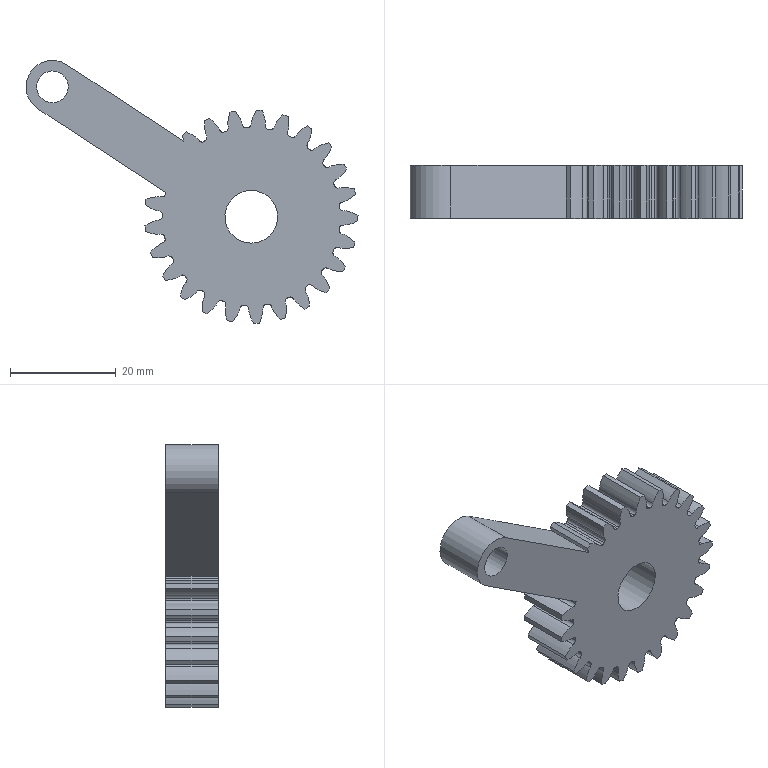Component | NX | JJZ-002 | 1 solid | 145 faces | volume 12845 mm3 | spline 115 | cylinder 26 | plane 4 | commonest cylinder face diameters 33.7 x23 10 x2 6 x1